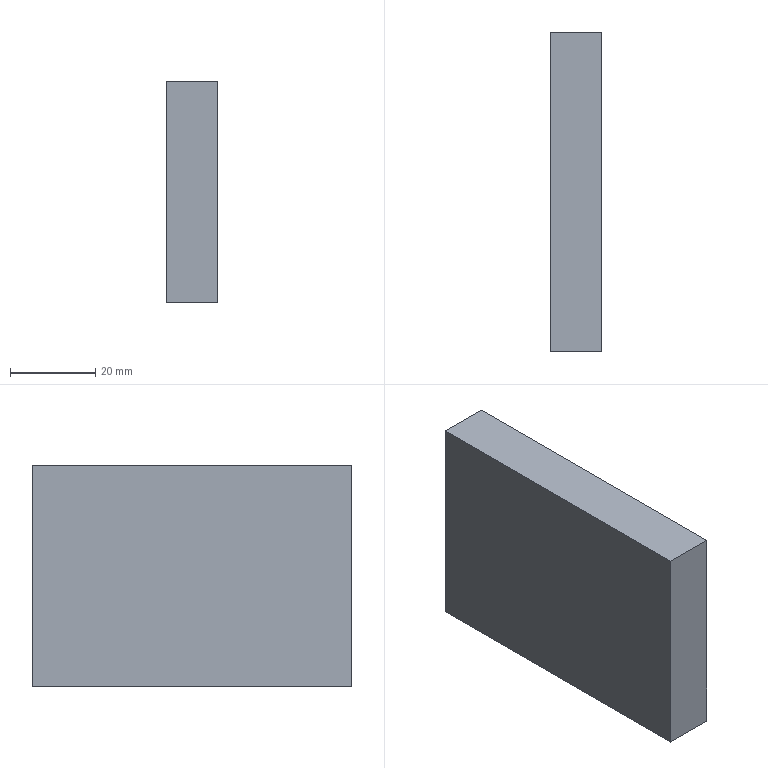Component | SolidWorks | BearingLiftingModule-1_RMT16X100S_0_+_CS1-G-2-1_CHEN123-AA-22-2 | 1 solid | 6 faces | box 12 x 75 x 52 mm | volume 46800 mm3 | plane 6
build123d program:
from build123d import *

# Parameters (mm, degrees)
SKETCH1_W           = 12
SKETCH1_H           = 75
BOSS_EXTRUDE1_DEPTH = 52


with BuildPart() as part:
    # Sketch1 → Boss-Extrude1 (new body)
    with BuildSketch(Plane.XY):
        Rectangle(SKETCH1_W, SKETCH1_H)
    extrude(amount=BOSS_EXTRUDE1_DEPTH)


solid = part.part

# Placed as in the assembly
solid = solid.moved(Location((121.999, -78.499, 10), (0, 0, 0)))
STEP:
#1=COLOUR_RGB('',0.7922,0.8196,0.9333);
#2=FILL_AREA_STYLE_COLOUR('',#1);
#3=FILL_AREA_STYLE('',(#2));
#4=SURFACE_STYLE_FILL_AREA(#3);
#5=SURFACE_SIDE_STYLE('',(#4));
#6=SURFACE_STYLE_USAGE(.BOTH.,#5);
#7=PRESENTATION_STYLE_ASSIGNMENT((#6));
#8=CARTESIAN_POINT('',(5.039,-4.567,0.3937));
#9=VERTEX_POINT('',#8);
#10=CARTESIAN_POINT('',(5.039,-1.614,0.3937));
#11=VERTEX_POINT('',#10);
#12=CARTESIAN_POINT('',(5.039,-4.567,0.3937));
#13=DIRECTION('',(0.,1.,0.));
#14=VECTOR('',#13,39.37);
#15=LINE('',#12,#14);
#16=EDGE_CURVE('',#9,#11,#15,.T.);
#17=ORIENTED_EDGE('',*,*,#16,.T.);
#18=CARTESIAN_POINT('',(5.039,-1.614,2.441));
#19=VERTEX_POINT('',#18);
#20=CARTESIAN_POINT('',(5.039,-1.614,2.441));
#21=DIRECTION('',(0.,0.,-1.));
#22=VECTOR('',#21,39.37);
#23=LINE('',#20,#22);
#24=EDGE_CURVE('',#19,#11,#23,.T.);
#25=ORIENTED_EDGE('',*,*,#24,.F.);
#26=CARTESIAN_POINT('',(5.039,-4.567,2.441));
#27=VERTEX_POINT('',#26);
#28=CARTESIAN_POINT('',(5.039,-4.567,2.441));
#29=DIRECTION('',(0.,1.,0.));
#30=VECTOR('',#29,39.37);
#31=LINE('',#28,#30);
#32=EDGE_CURVE('',#27,#19,#31,.T.);
#33=ORIENTED_EDGE('',*,*,#32,.F.);
#34=CARTESIAN_POINT('',(5.039,-4.567,2.441));
#35=DIRECTION('',(0.,0.,-1.));
#36=VECTOR('',#35,39.37);
#37=LINE('',#34,#36);
#38=EDGE_CURVE('',#27,#9,#37,.T.);
#39=ORIENTED_EDGE('',*,*,#38,.T.);
#40=EDGE_LOOP('',(#17,#25,#33,#39));
#41=FACE_OUTER_BOUND('',#40,.T.);
#42=CARTESIAN_POINT('',(5.039,-4.567,2.441));
#43=DIRECTION('',(-1.,0.,0.));
#44=DIRECTION('',(0.,0.,1.));
#45=AXIS2_PLACEMENT_3D('',#42,#43,#44);
#46=PLANE('',#45);
#47=ADVANCED_FACE('',(#41),#46,.F.);
#48=CARTESIAN_POINT('',(4.567,-1.614,0.3937));
#49=VERTEX_POINT('',#48);
#50=CARTESIAN_POINT('',(4.567,-1.614,0.3937));
#51=DIRECTION('',(-1.,0.,0.));
#52=VECTOR('',#51,39.37);
#53=LINE('',#50,#52);
#54=EDGE_CURVE('',#11,#49,#53,.T.);
#55=ORIENTED_EDGE('',*,*,#54,.T.);
#56=CARTESIAN_POINT('',(4.567,-1.614,2.441));
#57=VERTEX_POINT('',#56);
#58=CARTESIAN_POINT('',(4.567,-1.614,2.441));
#59=DIRECTION('',(0.,0.,-1.));
#60=VECTOR('',#59,39.37);
#61=LINE('',#58,#60);
#62=EDGE_CURVE('',#57,#49,#61,.T.);
#63=ORIENTED_EDGE('',*,*,#62,.F.);
#64=CARTESIAN_POINT('',(4.567,-1.614,2.441));
#65=DIRECTION('',(-1.,0.,0.));
#66=VECTOR('',#65,39.37);
#67=LINE('',#64,#66);
#68=EDGE_CURVE('',#19,#57,#67,.T.);
#69=ORIENTED_EDGE('',*,*,#68,.F.);
#70=ORIENTED_EDGE('',*,*,#24,.T.);
#71=EDGE_LOOP('',(#55,#63,#69,#70));
#72=FACE_OUTER_BOUND('',#71,.T.);
#73=CARTESIAN_POINT('',(4.567,-1.614,2.441));
#74=DIRECTION('',(0.,-1.,0.));
#75=DIRECTION('',(0.,0.,-1.));
#76=AXIS2_PLACEMENT_3D('',#73,#74,#75);
#77=PLANE('',#76);
#78=ADVANCED_FACE('',(#72),#77,.F.);
#79=CARTESIAN_POINT('',(4.567,-4.567,0.3937));
#80=VERTEX_POINT('',#79);
#81=CARTESIAN_POINT('',(4.567,-4.567,0.3937));
#82=DIRECTION('',(0.,-1.,0.));
#83=VECTOR('',#82,39.37);
#84=LINE('',#81,#83);
#85=EDGE_CURVE('',#49,#80,#84,.T.);
#86=ORIENTED_EDGE('',*,*,#85,.T.);
#87=CARTESIAN_POINT('',(4.567,-4.567,2.441));
#88=VERTEX_POINT('',#87);
#89=CARTESIAN_POINT('',(4.567,-4.567,2.441));
#90=DIRECTION('',(0.,0.,-1.));
#91=VECTOR('',#90,39.37);
#92=LINE('',#89,#91);
#93=EDGE_CURVE('',#88,#80,#92,.T.);
#94=ORIENTED_EDGE('',*,*,#93,.F.);
#95=CARTESIAN_POINT('',(4.567,-4.567,2.441));
#96=DIRECTION('',(0.,-1.,0.));
#97=VECTOR('',#96,39.37);
#98=LINE('',#95,#97);
#99=EDGE_CURVE('',#57,#88,#98,.T.);
#100=ORIENTED_EDGE('',*,*,#99,.F.);
#101=ORIENTED_EDGE('',*,*,#62,.T.);
#102=EDGE_LOOP('',(#86,#94,#100,#101));
#103=FACE_OUTER_BOUND('',#102,.T.);
#104=CARTESIAN_POINT('',(4.567,-4.567,2.441));
#105=DIRECTION('',(1.,0.,0.));
#106=DIRECTION('',(0.,0.,-1.));
#107=AXIS2_PLACEMENT_3D('',#104,#105,#106);
#108=PLANE('',#107);
#109=ADVANCED_FACE('',(#103),#108,.F.);
#110=CARTESIAN_POINT('',(4.567,-4.567,0.3937));
#111=DIRECTION('',(1.,0.,0.));
#112=VECTOR('',#111,39.37);
#113=LINE('',#110,#112);
#114=EDGE_CURVE('',#80,#9,#113,.T.);
#115=ORIENTED_EDGE('',*,*,#114,.T.);
#116=ORIENTED_EDGE('',*,*,#38,.F.);
#117=CARTESIAN_POINT('',(4.567,-4.567,2.441));
#118=DIRECTION('',(1.,0.,0.));
#119=VECTOR('',#118,39.37);
#120=LINE('',#117,#119);
#121=EDGE_CURVE('',#88,#27,#120,.T.);
#122=ORIENTED_EDGE('',*,*,#121,.F.);
#123=ORIENTED_EDGE('',*,*,#93,.T.);
#124=EDGE_LOOP('',(#115,#116,#122,#123));
#125=FACE_OUTER_BOUND('',#124,.T.);
#126=CARTESIAN_POINT('',(4.567,-4.567,2.441));
#127=DIRECTION('',(0.,1.,0.));
#128=DIRECTION('',(0.,0.,1.));
#129=AXIS2_PLACEMENT_3D('',#126,#127,#128);
#130=PLANE('',#129);
#131=ADVANCED_FACE('',(#125),#130,.F.);
#132=ORIENTED_EDGE('',*,*,#32,.T.);
#133=ORIENTED_EDGE('',*,*,#68,.T.);
#134=ORIENTED_EDGE('',*,*,#99,.T.);
#135=ORIENTED_EDGE('',*,*,#121,.T.);
#136=EDGE_LOOP('',(#132,#133,#134,#135));
#137=FACE_OUTER_BOUND('',#136,.T.);
#138=CARTESIAN_POINT('',(4.803,-3.091,2.441));
#139=DIRECTION('',(0.,0.,-1.));
#140=DIRECTION('',(-1.,0.,0.));
#141=AXIS2_PLACEMENT_3D('',#138,#139,#140);
#142=PLANE('',#141);
#143=ADVANCED_FACE('',(#137),#142,.F.);
#144=ORIENTED_EDGE('',*,*,#16,.F.);
#145=ORIENTED_EDGE('',*,*,#114,.F.);
#146=ORIENTED_EDGE('',*,*,#85,.F.);
#147=ORIENTED_EDGE('',*,*,#54,.F.);
#148=EDGE_LOOP('',(#144,#145,#146,#147));
#149=FACE_OUTER_BOUND('',#148,.T.);
#150=CARTESIAN_POINT('',(4.803,-3.091,0.3937));
#151=DIRECTION('',(0.,0.,-1.));
#152=DIRECTION('',(-1.,0.,0.));
#153=AXIS2_PLACEMENT_3D('',#150,#151,#152);
#154=PLANE('',#153);
#155=ADVANCED_FACE('',(#149),#154,.T.);
#156=CLOSED_SHELL('',(#47,#78,#109,#131,#143,#155));
#157=MANIFOLD_SOLID_BREP('',#156);
#158=STYLED_ITEM('',(#7),#157);
#159=(LENGTH_UNIT()NAMED_UNIT(*)SI_UNIT($,.METRE.));
#160=LENGTH_MEASURE_WITH_UNIT(LENGTH_MEASURE(0.0254),#159);
#161=DIMENSIONAL_EXPONENTS(1.,0.,0.,0.,0.,0.,0.);
#162=(CONVERSION_BASED_UNIT('',#160)LENGTH_UNIT()NAMED_UNIT(#161));
#163=UNCERTAINTY_MEASURE_WITH_UNIT(LENGTH_MEASURE(0.00001),#162,'','');
#164=(NAMED_UNIT(*)PLANE_ANGLE_UNIT()SI_UNIT($,.RADIAN.));
#165=(NAMED_UNIT(*)SI_UNIT($,.STERADIAN.)SOLID_ANGLE_UNIT());
#166=(GEOMETRIC_REPRESENTATION_CONTEXT(3)GLOBAL_UNCERTAINTY_ASSIGNED_CONTEXT((#163))GLOBAL_UNIT_ASSIGNED_CONTEXT((#162,#164,#165))REPRESENTATION_CONTEXT('',''));
#167=MECHANICAL_DESIGN_GEOMETRIC_PRESENTATION_REPRESENTATION('',(#158),#166);
#168=CARTESIAN_POINT('',(0.,0.,0.));
#169=DIRECTION('',(0.,0.,1.));
#170=DIRECTION('',(1.,0.,0.));
#171=AXIS2_PLACEMENT_3D('',#168,#169,#170);
#172=(LENGTH_UNIT()NAMED_UNIT(*)SI_UNIT($,.METRE.));
#173=LENGTH_MEASURE_WITH_UNIT(LENGTH_MEASURE(0.0254),#172);
#174=DIMENSIONAL_EXPONENTS(1.,0.,0.,0.,0.,0.,0.);
#175=(CONVERSION_BASED_UNIT('',#173)LENGTH_UNIT()NAMED_UNIT(#174));
#176=UNCERTAINTY_MEASURE_WITH_UNIT(LENGTH_MEASURE(0.00001),#175,'','');
#177=(NAMED_UNIT(*)PLANE_ANGLE_UNIT()SI_UNIT($,.RADIAN.));
#178=(NAMED_UNIT(*)SI_UNIT($,.STERADIAN.)SOLID_ANGLE_UNIT());
#179=(GEOMETRIC_REPRESENTATION_CONTEXT(3)GLOBAL_UNCERTAINTY_ASSIGNED_CONTEXT((#176))GLOBAL_UNIT_ASSIGNED_CONTEXT((#175,#177,#178))REPRESENTATION_CONTEXT('',''));
#180=ADVANCED_BREP_SHAPE_REPRESENTATION('',(#157,#171),#179);
#181=PRESENTATION_LAYER_ASSIGNMENT('','',(#158));